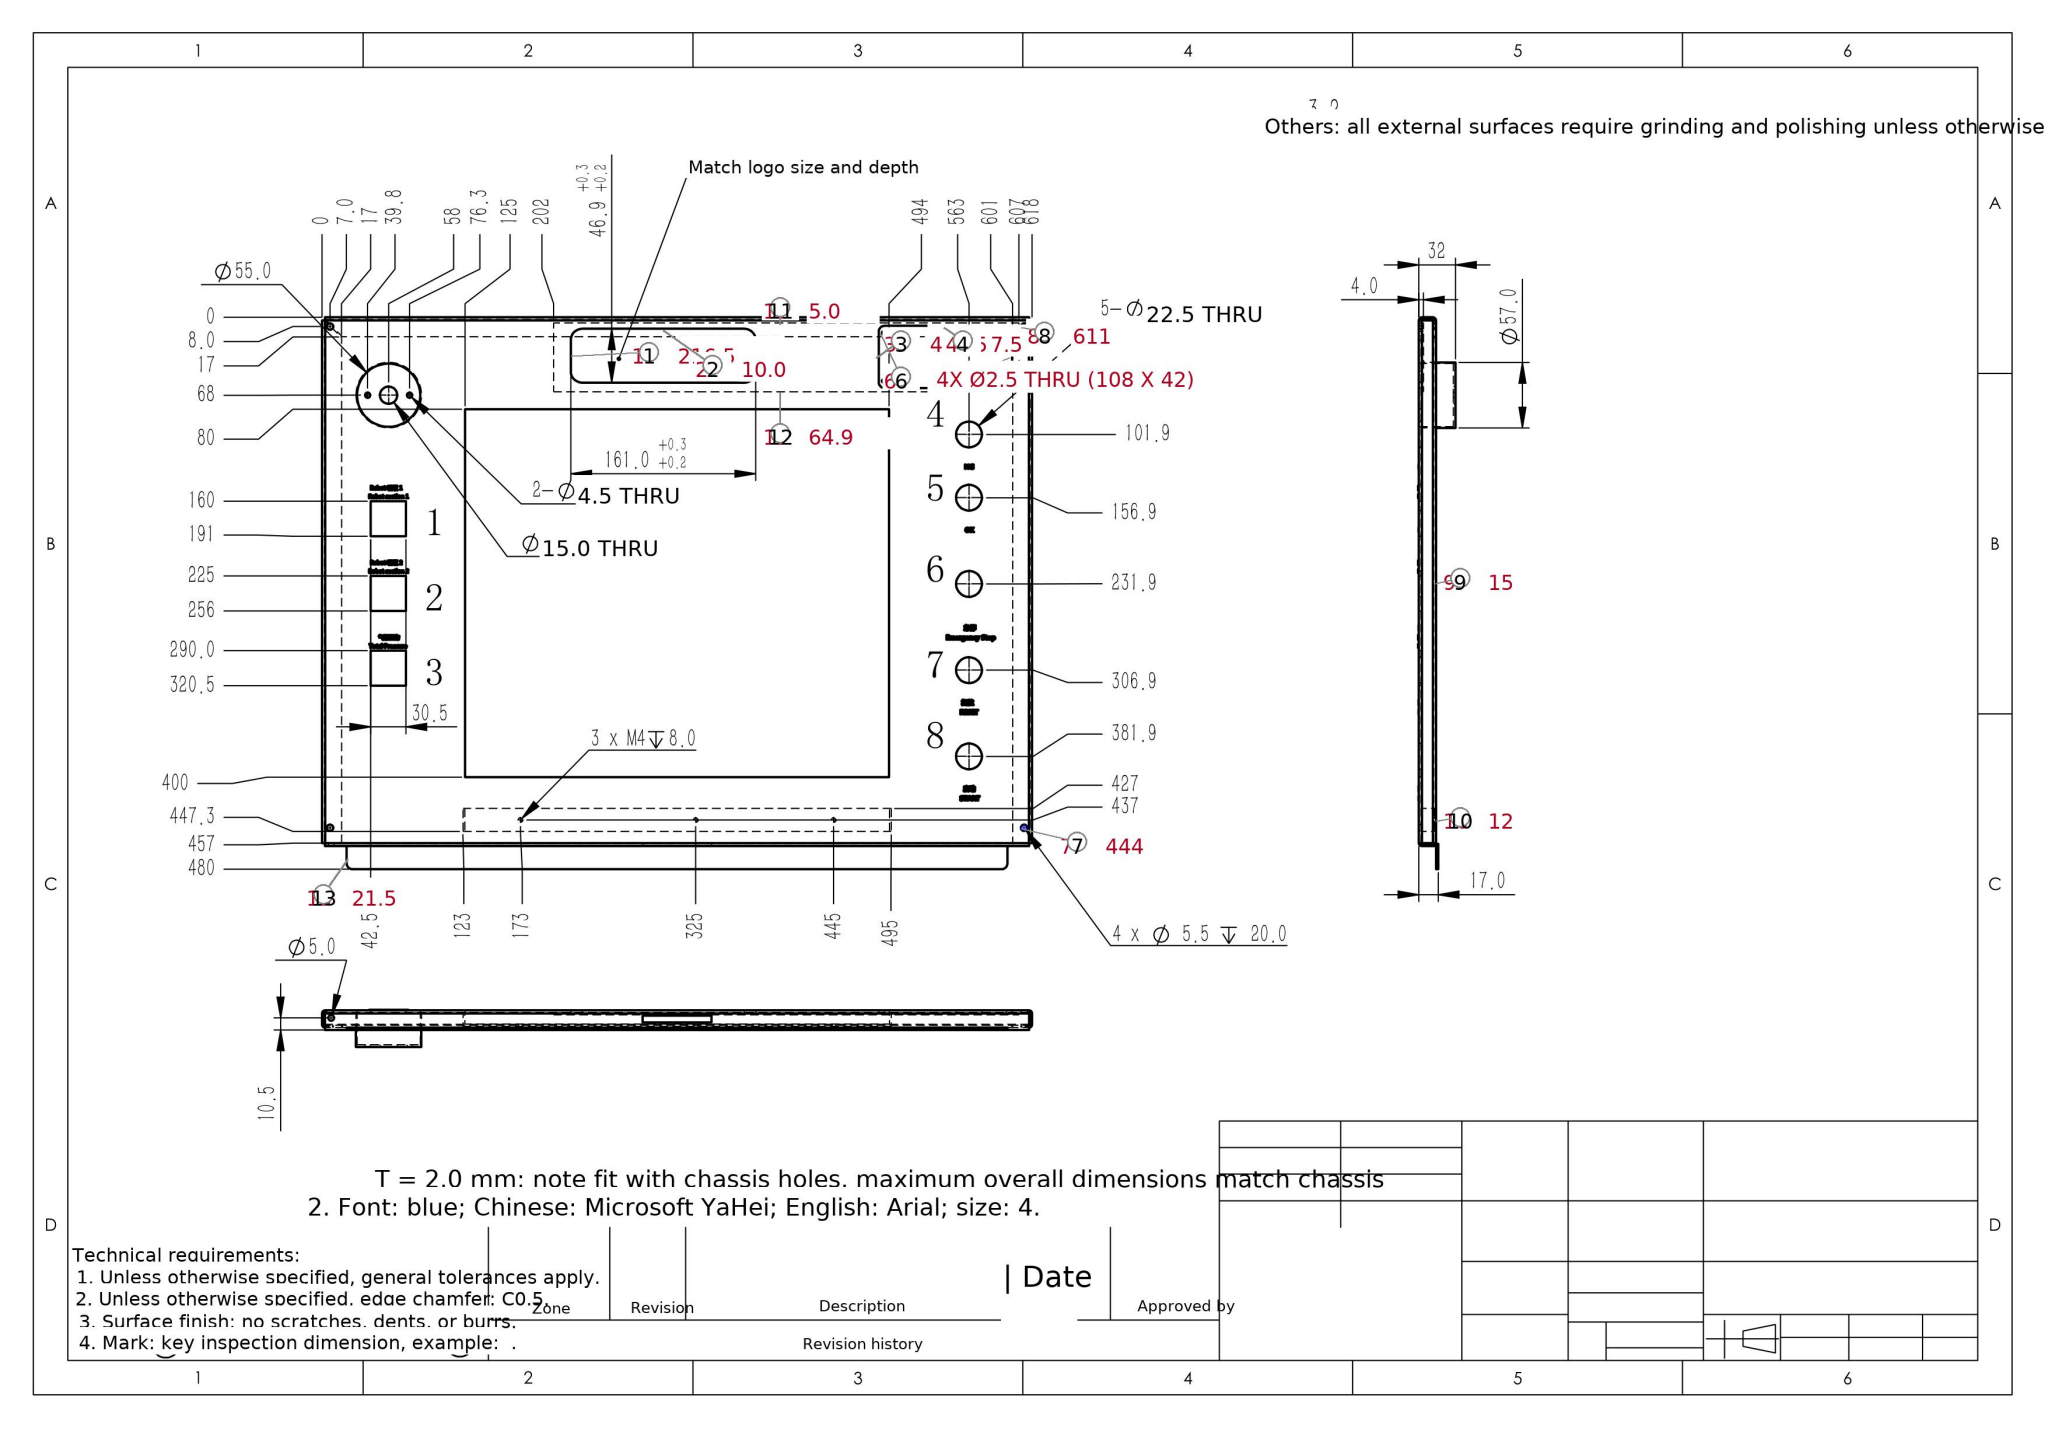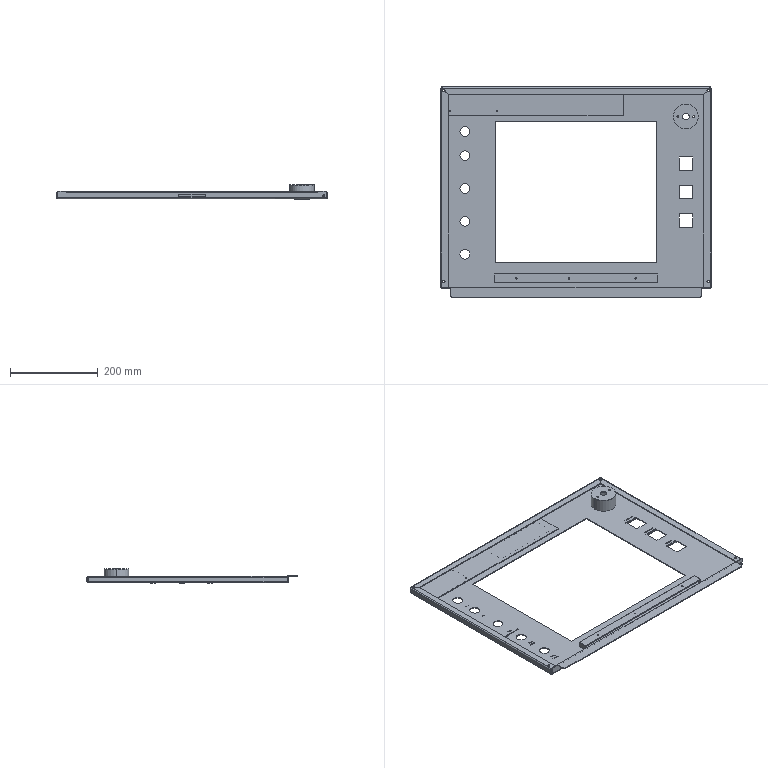Part | SolidWorks | mm | 1 solid | 1835 faces | box 618 x 480 x 32.5 mm | volume 483394 mm3 | plane 1104 | spline 653 | cylinder 78 | commonest cylinder face diameters 5.5 x18 22.5 x10 2.5 x8 5.473 x7 1.473 x7 3.3 x6 10 x6 4.5 x4